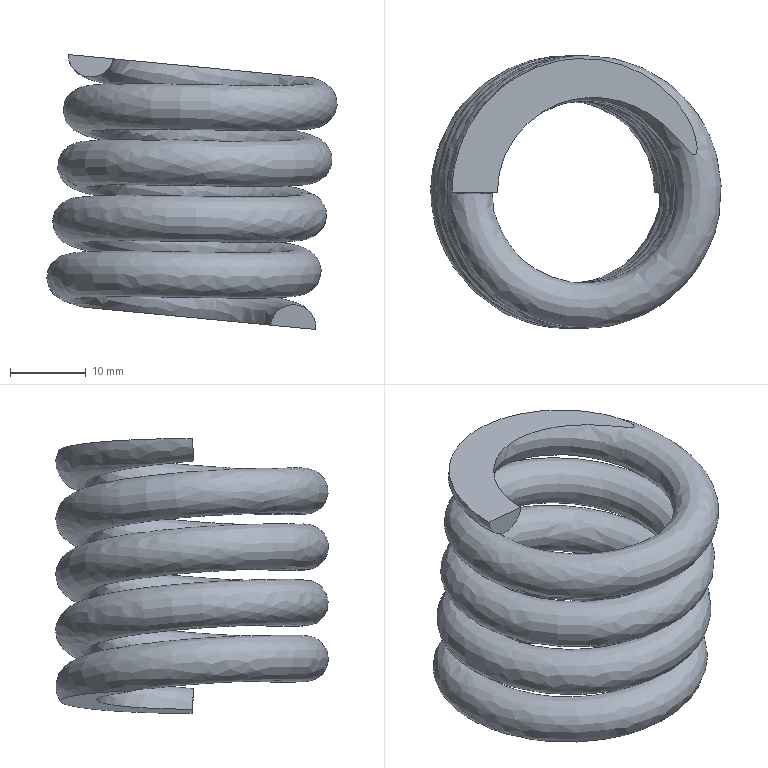Component | NX | YANHUANG | 1 solid | 5 faces | volume 11518 mm3 | plane 4 | spline 1